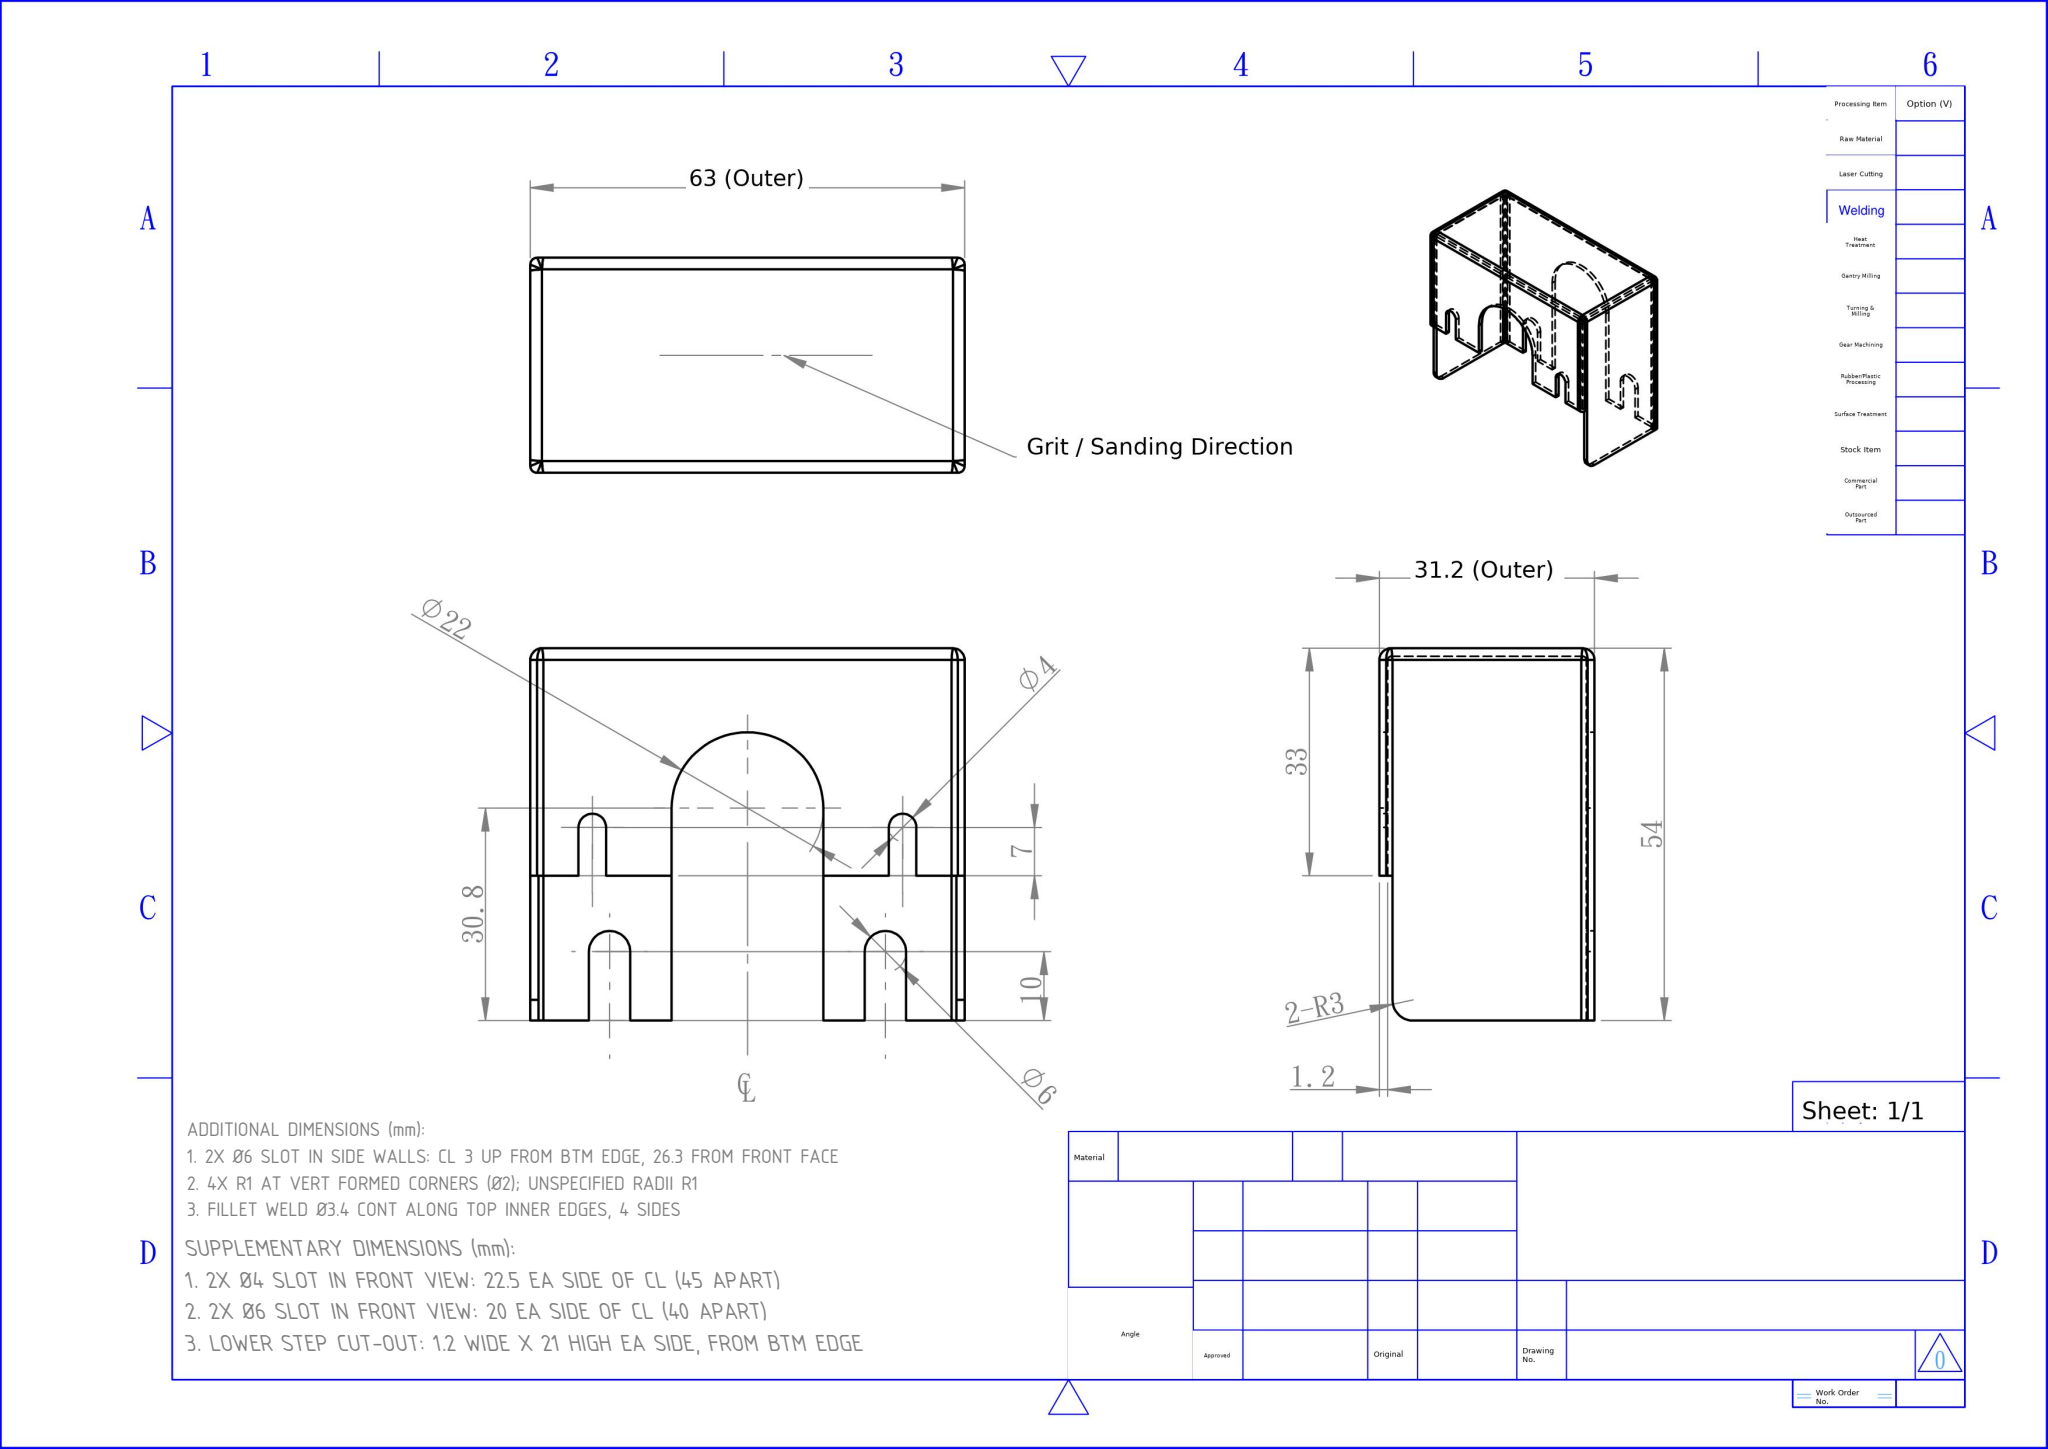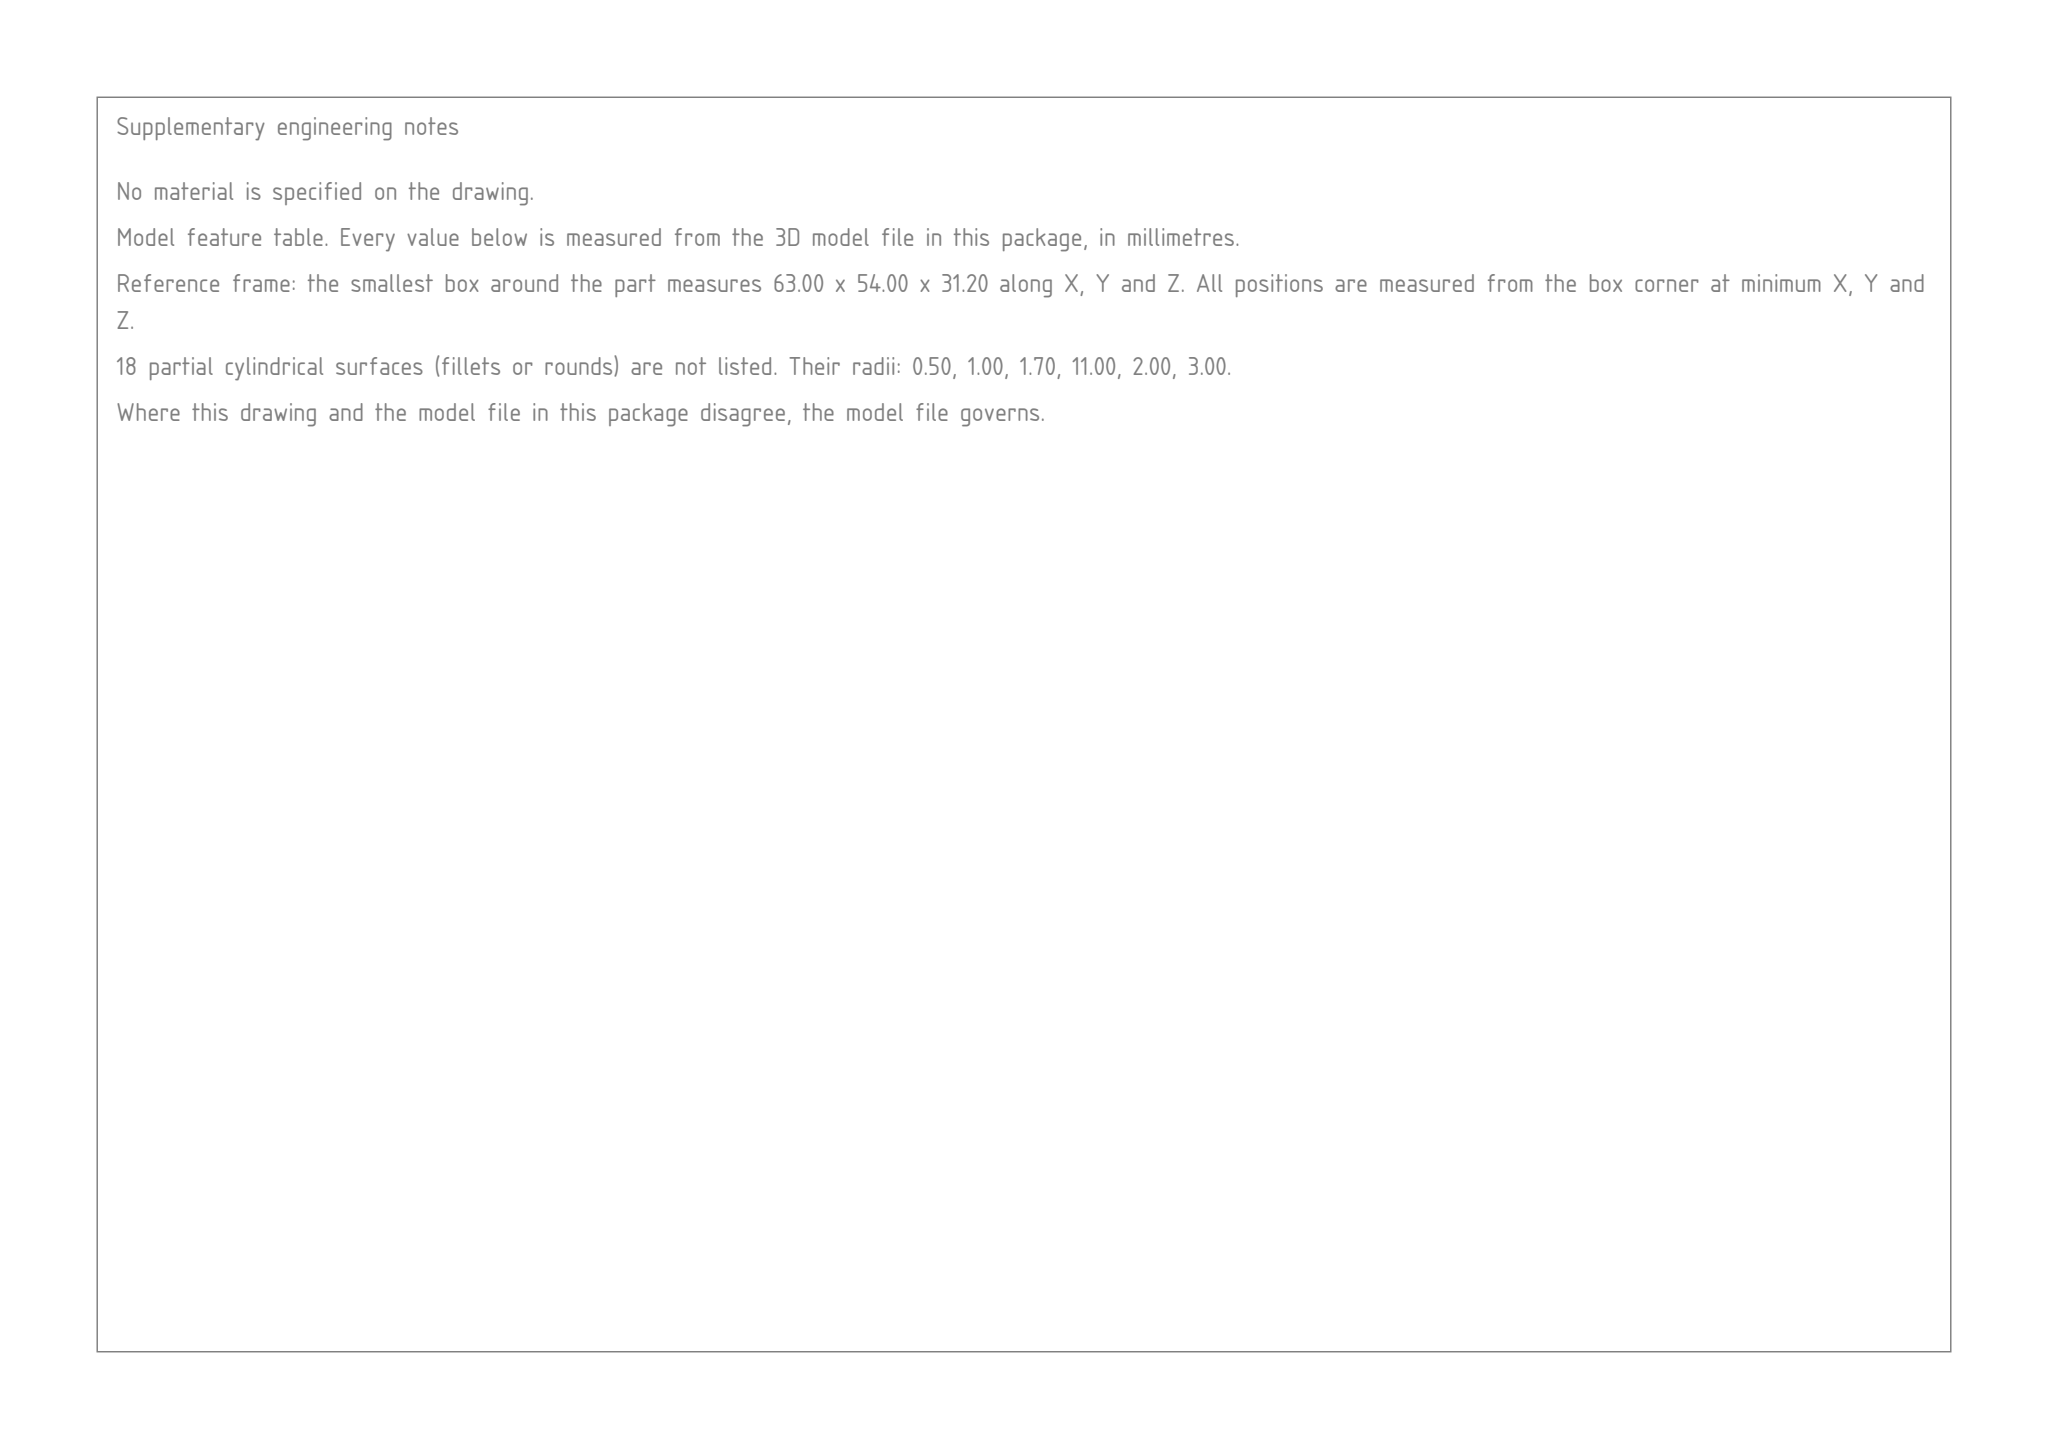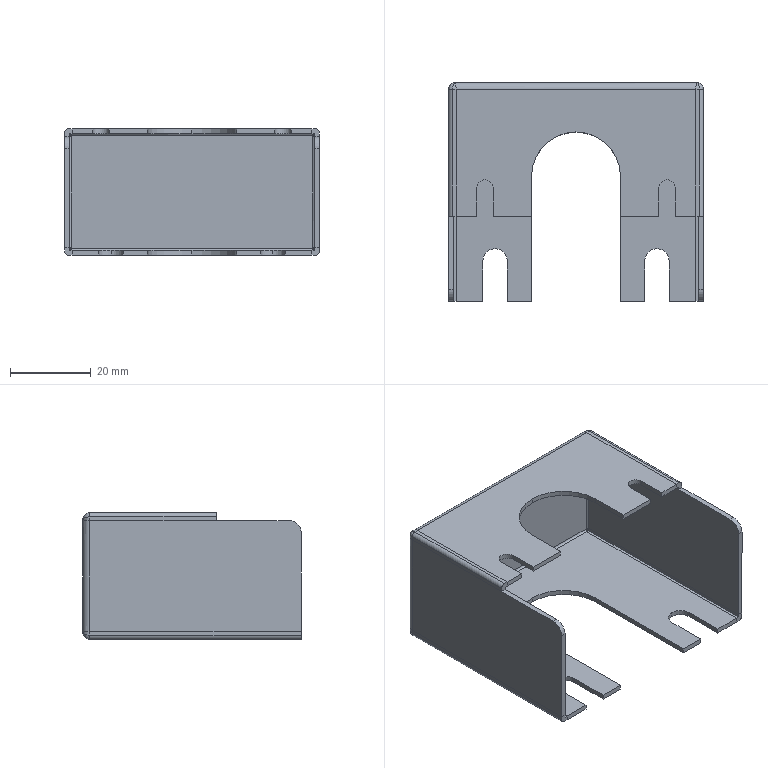Part | SolidWorks | mm | 1 solid | 98 faces | box 63 x 54 x 31.2 mm | volume 10434 mm3 | plane 54 | cylinder 24 | spline 20 | commonest cylinder face diameters 6 x6 22 x4 3.4 x4 1 x4 2 x4 4 x2